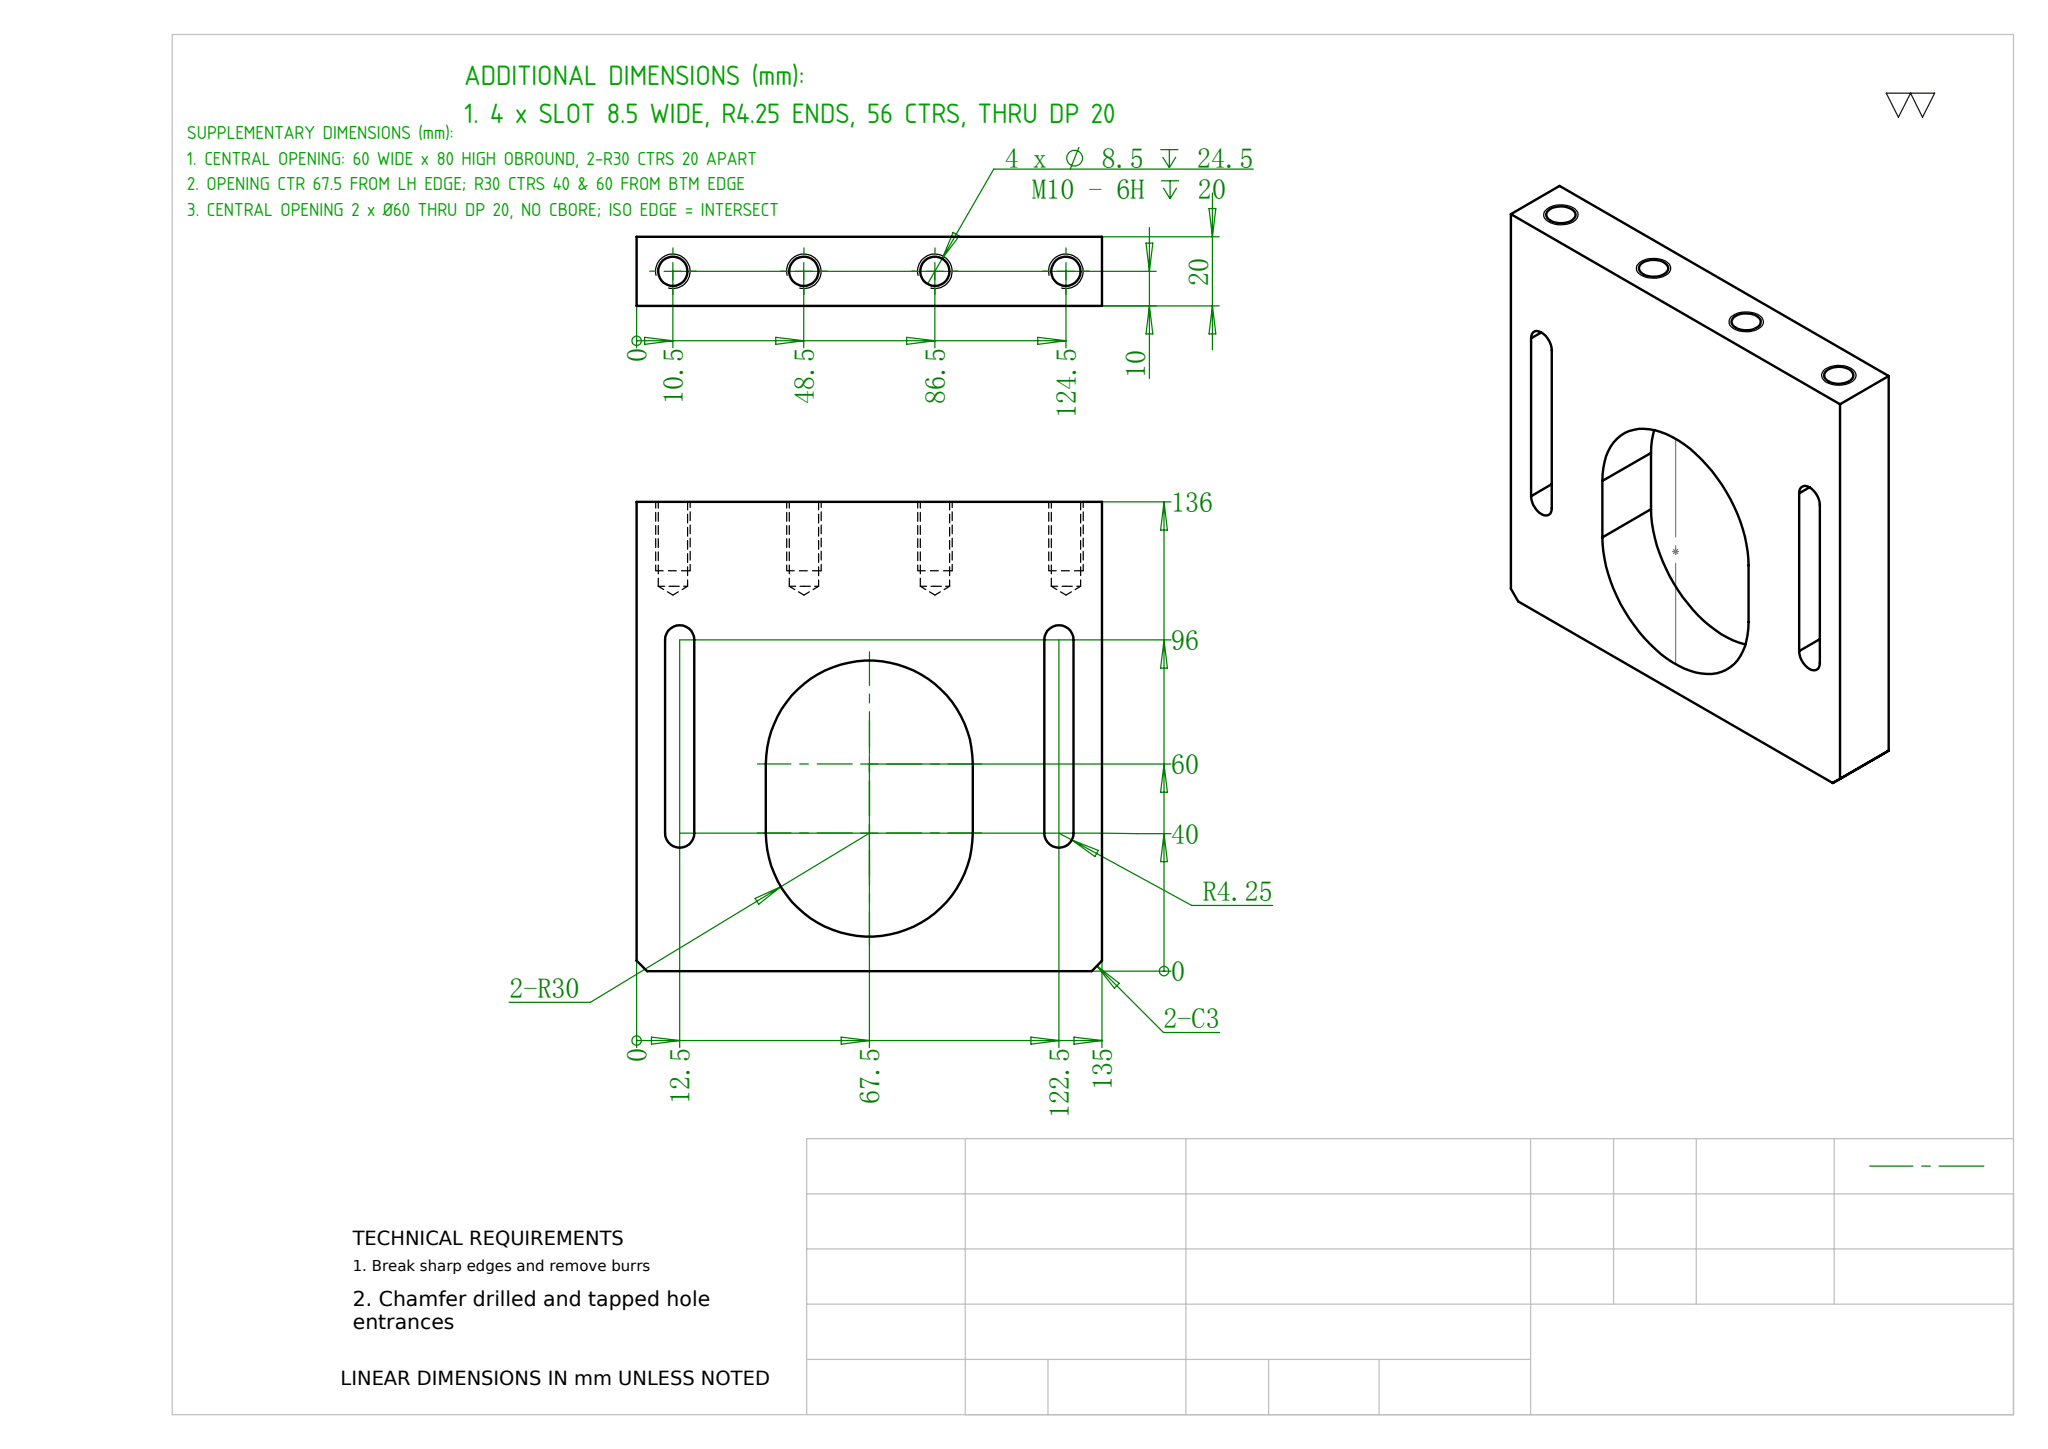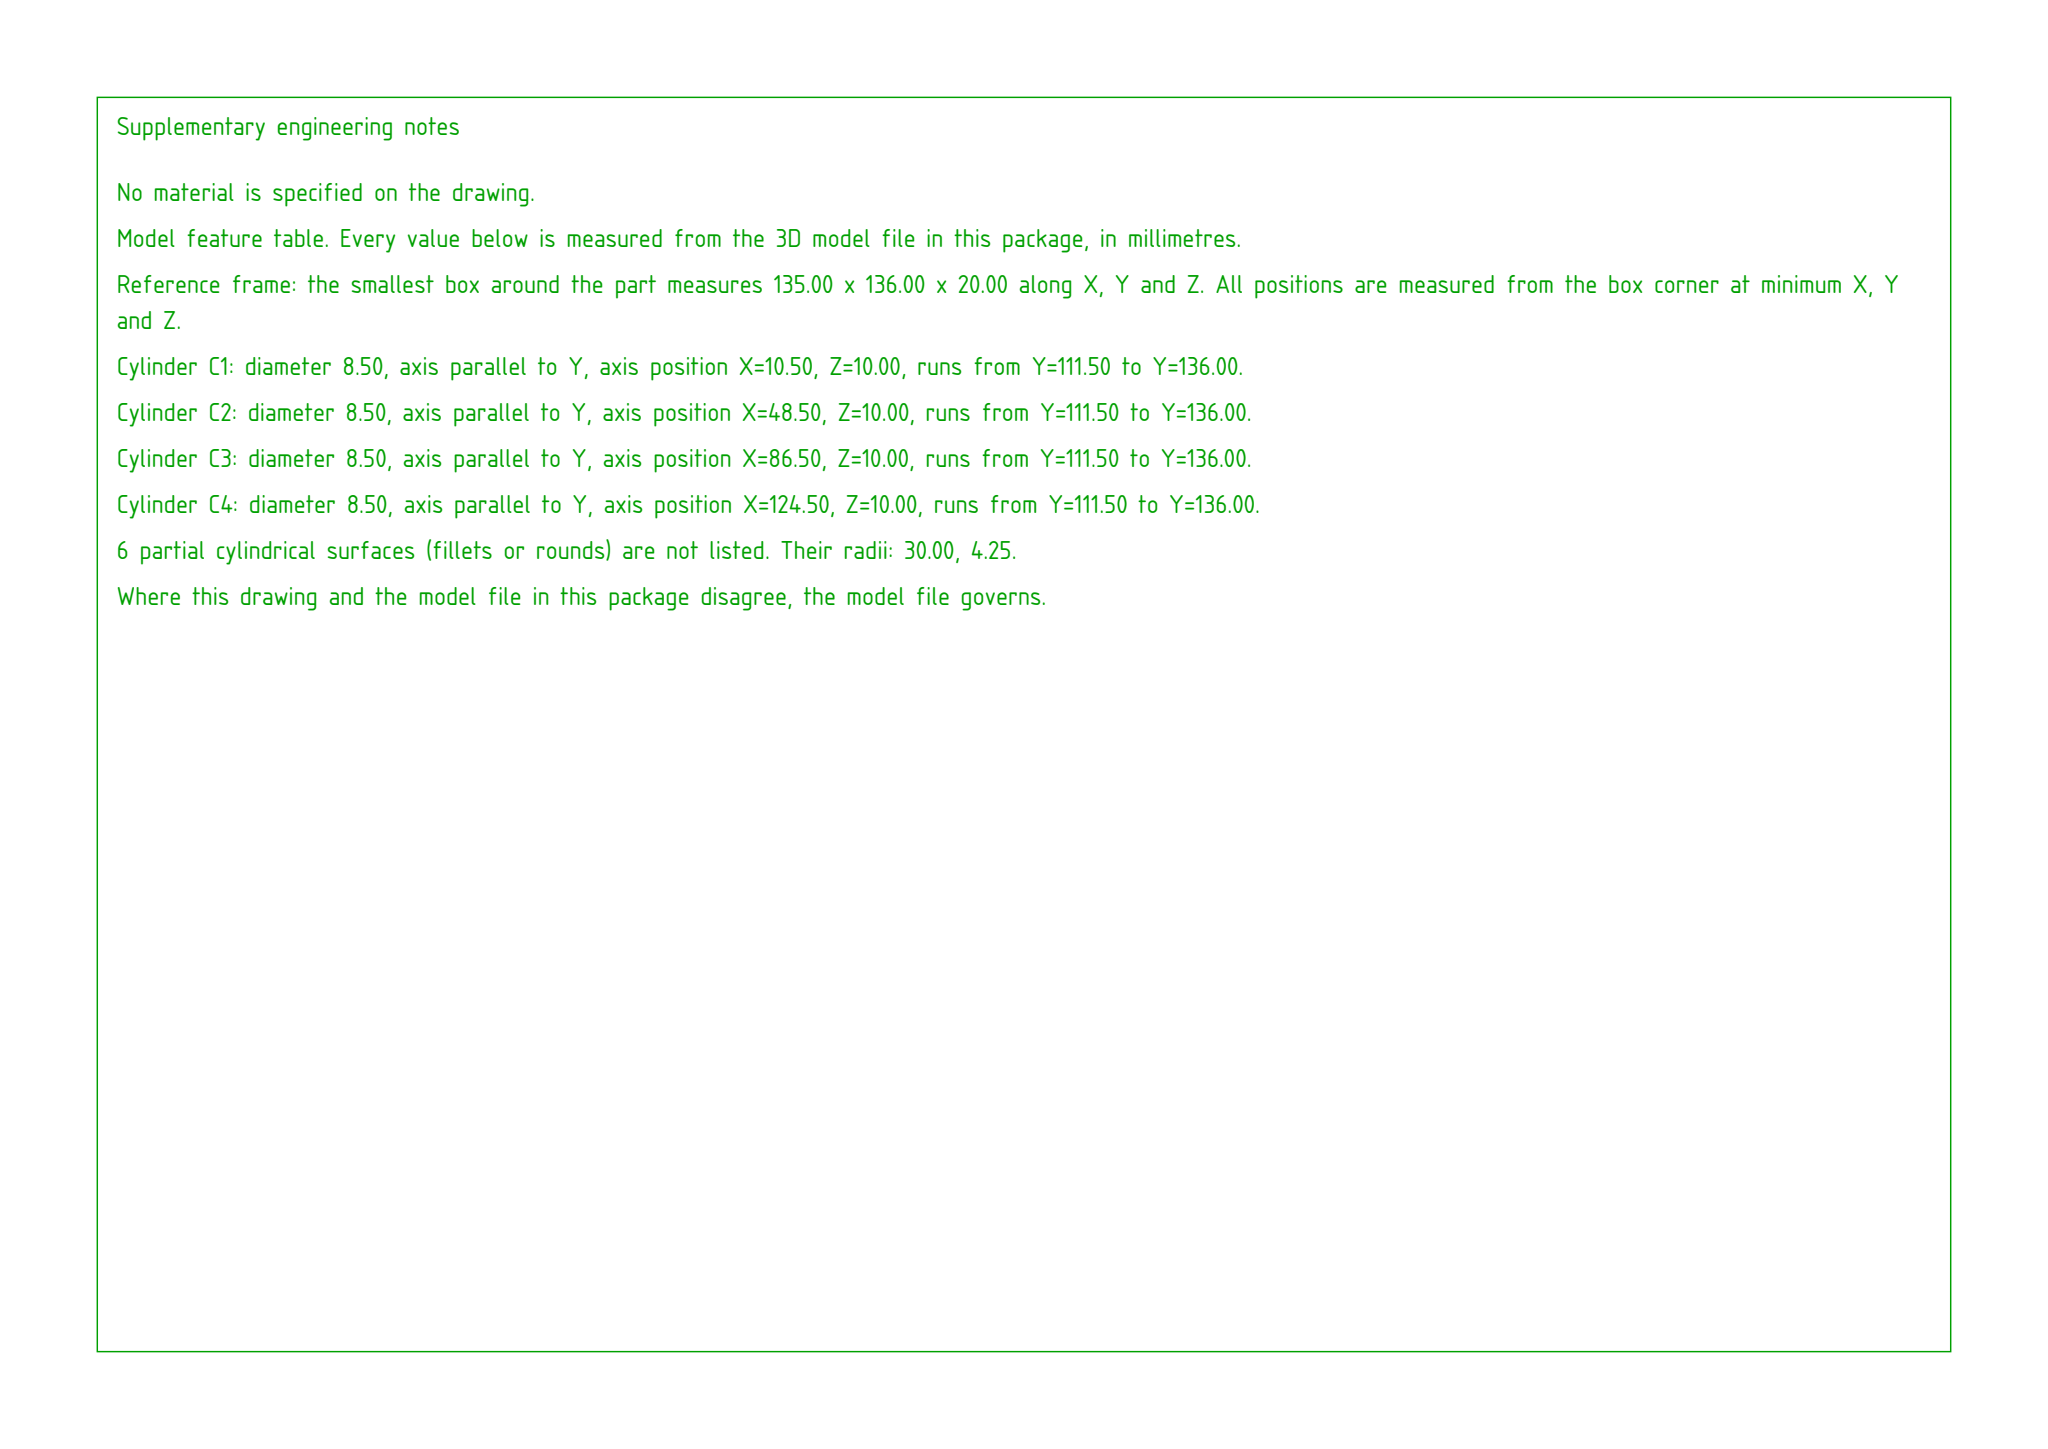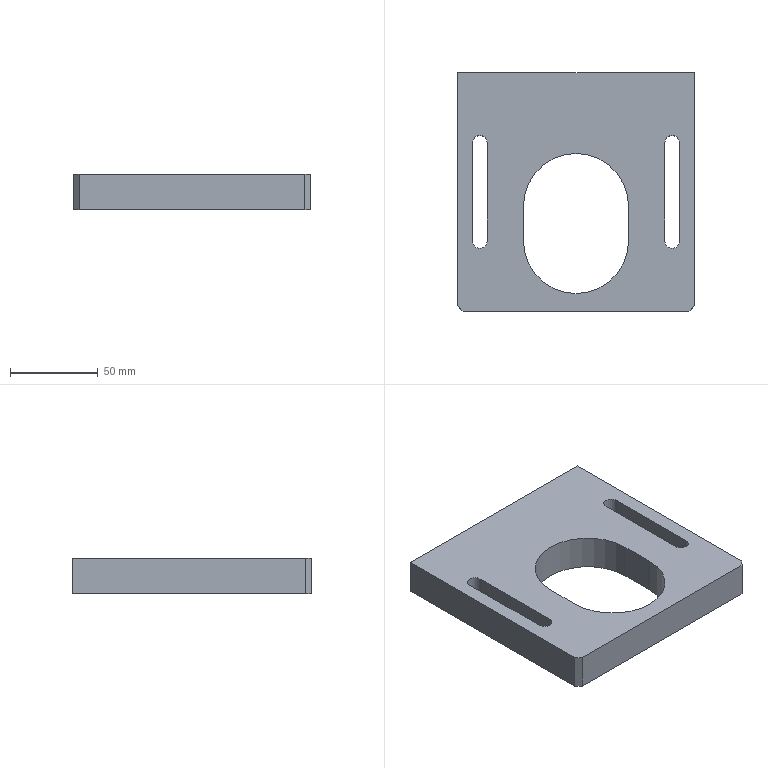Part | SolidWorks | mm | 1 solid | 36 faces | box 135 x 136 x 20 mm | volume 259407 mm3 | cylinder 14 | plane 14 | cone 8 | commonest cylinder face diameters 8.5 x12 60 x2